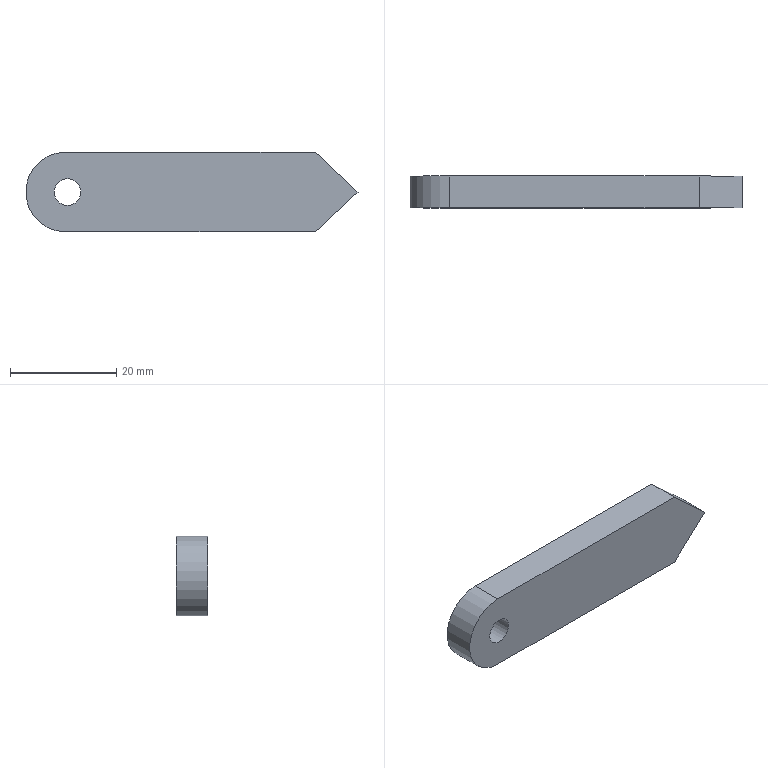Component | NX | TRI_SLIDER_2 | 1 solid | 8 faces | box 62.5 x 6 x 15 mm | volume 5000 mm3 | plane 6 | cylinder 2 | commonest cylinder face diameters 15 x1 5 x1
STEP:
#1=CARTESIAN_POINT('',(0.,0.,0.));
#2=DIRECTION('',(0.,0.,1.));
#3=DIRECTION('',(1.,0.,0.));
#4=AXIS2_PLACEMENT_3D('',#1,#2,#3);
#5=CARTESIAN_POINT('',(54.023,-12.,79.479));
#6=VERTEX_POINT('',#5);
#7=CARTESIAN_POINT('',(46.003,-12.,72.));
#8=VERTEX_POINT('',#7);
#9=CARTESIAN_POINT('',(54.023,-12.,79.479));
#10=DIRECTION('',(-0.7314,0.,-0.682));
#11=VECTOR('',#10,1.);
#12=LINE('',#9,#11);
#13=CARTESIAN_POINT('',(54.023,-18.,79.479));
#14=DIRECTION('',(0.682,0.,-0.7314));
#15=DIRECTION('',(0.7314,0.,0.682));
#16=AXIS2_PLACEMENT_3D('',#13,#14,#15);
#17=PLANE('',#16);
#18=CARTESIAN_POINT('',(0.,-6.));
#19=DIRECTION('',(-1.,0.));
#20=VECTOR('',#19,1.);
#21=LINE('',#18,#20);
#22=(GEOMETRIC_REPRESENTATION_CONTEXT(2)PARAMETRIC_REPRESENTATION_CONTEXT()REPRESENTATION_CONTEXT('',''));
#23=DEFINITIONAL_REPRESENTATION('',(#21),#22);
#24=PCURVE('',#17,#23);
#25=CARTESIAN_POINT('',(-0.9773,-12.,79.5));
#26=DIRECTION('',(0.,1.,0.));
#27=DIRECTION('',(1.,0.,0.));
#28=AXIS2_PLACEMENT_3D('',#25,#26,#27);
#29=PLANE('',#28);
#30=CARTESIAN_POINT('',(55.,0.02132));
#31=DIRECTION('',(-0.7314,0.682));
#32=VECTOR('',#31,1.);
#33=LINE('',#30,#32);
#34=(GEOMETRIC_REPRESENTATION_CONTEXT(2)PARAMETRIC_REPRESENTATION_CONTEXT()REPRESENTATION_CONTEXT('',''));
#35=DEFINITIONAL_REPRESENTATION('',(#33),#34);
#36=PCURVE('',#29,#35);
#37=SURFACE_CURVE('',#12,(#24,#36),.PCURVE_S1.);
#38=EDGE_CURVE('',#6,#8,#37,.T.);
#39=ORIENTED_EDGE('',*,*,#38,.F.);
#40=CARTESIAN_POINT('',(54.023,-18.,79.479));
#41=VERTEX_POINT('',#40);
#42=CARTESIAN_POINT('',(54.023,-18.,79.479));
#43=DIRECTION('',(0.,1.,0.));
#44=VECTOR('',#43,1.);
#45=LINE('',#42,#44);
#46=CARTESIAN_POINT('',(0.,0.));
#47=DIRECTION('',(0.,-1.));
#48=VECTOR('',#47,1.);
#49=LINE('',#46,#48);
#50=(GEOMETRIC_REPRESENTATION_CONTEXT(2)PARAMETRIC_REPRESENTATION_CONTEXT()REPRESENTATION_CONTEXT('',''));
#51=DEFINITIONAL_REPRESENTATION('',(#49),#50);
#52=PCURVE('',#17,#51);
#53=CARTESIAN_POINT('',(45.957,-18.,87.));
#54=DIRECTION('',(0.682,0.,0.7314));
#55=DIRECTION('',(-0.7314,0.,0.682));
#56=AXIS2_PLACEMENT_3D('',#53,#54,#55);
#57=PLANE('',#56);
#58=CARTESIAN_POINT('',(-11.028,0.));
#59=DIRECTION('',(0.,-1.));
#60=VECTOR('',#59,1.);
#61=LINE('',#58,#60);
#62=(GEOMETRIC_REPRESENTATION_CONTEXT(2)PARAMETRIC_REPRESENTATION_CONTEXT()REPRESENTATION_CONTEXT('',''));
#63=DEFINITIONAL_REPRESENTATION('',(#61),#62);
#64=PCURVE('',#57,#63);
#65=SURFACE_CURVE('',#45,(#52,#64),.PCURVE_S1.);
#66=EDGE_CURVE('',#41,#6,#65,.T.);
#67=ORIENTED_EDGE('',*,*,#66,.F.);
#68=CARTESIAN_POINT('',(46.003,-18.,72.));
#69=VERTEX_POINT('',#68);
#70=CARTESIAN_POINT('',(54.023,-18.,79.479));
#71=DIRECTION('',(-0.7314,0.,-0.682));
#72=VECTOR('',#71,1.);
#73=LINE('',#70,#72);
#74=CARTESIAN_POINT('',(0.,0.));
#75=DIRECTION('',(-1.,0.));
#76=VECTOR('',#75,1.);
#77=LINE('',#74,#76);
#78=(GEOMETRIC_REPRESENTATION_CONTEXT(2)PARAMETRIC_REPRESENTATION_CONTEXT()REPRESENTATION_CONTEXT('',''));
#79=DEFINITIONAL_REPRESENTATION('',(#77),#78);
#80=PCURVE('',#17,#79);
#81=CARTESIAN_POINT('',(-0.9773,-18.,79.5));
#82=DIRECTION('',(0.,1.,0.));
#83=DIRECTION('',(1.,0.,0.));
#84=AXIS2_PLACEMENT_3D('',#81,#82,#83);
#85=PLANE('',#84);
#86=CARTESIAN_POINT('',(55.,0.02132));
#87=DIRECTION('',(-0.7314,0.682));
#88=VECTOR('',#87,1.);
#89=LINE('',#86,#88);
#90=(GEOMETRIC_REPRESENTATION_CONTEXT(2)PARAMETRIC_REPRESENTATION_CONTEXT()REPRESENTATION_CONTEXT('',''));
#91=DEFINITIONAL_REPRESENTATION('',(#89),#90);
#92=PCURVE('',#85,#91);
#93=SURFACE_CURVE('',#73,(#80,#92),.PCURVE_S1.);
#94=EDGE_CURVE('',#41,#69,#93,.T.);
#95=ORIENTED_EDGE('',*,*,#94,.T.);
#96=CARTESIAN_POINT('',(46.003,-18.,72.));
#97=DIRECTION('',(0.,1.,0.));
#98=VECTOR('',#97,1.);
#99=LINE('',#96,#98);
#100=CARTESIAN_POINT('',(-10.966,0.));
#101=DIRECTION('',(0.,-1.));
#102=VECTOR('',#101,1.);
#103=LINE('',#100,#102);
#104=(GEOMETRIC_REPRESENTATION_CONTEXT(2)PARAMETRIC_REPRESENTATION_CONTEXT()REPRESENTATION_CONTEXT('',''));
#105=DEFINITIONAL_REPRESENTATION('',(#103),#104);
#106=PCURVE('',#17,#105);
#107=CARTESIAN_POINT('',(46.003,-18.,72.));
#108=DIRECTION('',(0.,0.,-1.));
#109=DIRECTION('',(1.,0.,0.));
#110=AXIS2_PLACEMENT_3D('',#107,#108,#109);
#111=PLANE('',#110);
#112=CARTESIAN_POINT('',(0.,0.));
#113=DIRECTION('',(0.,-1.));
#114=VECTOR('',#113,1.);
#115=LINE('',#112,#114);
#116=(GEOMETRIC_REPRESENTATION_CONTEXT(2)PARAMETRIC_REPRESENTATION_CONTEXT()REPRESENTATION_CONTEXT('',''));
#117=DEFINITIONAL_REPRESENTATION('',(#115),#116);
#118=PCURVE('',#111,#117);
#119=SURFACE_CURVE('',#99,(#106,#118),.PCURVE_S1.);
#120=EDGE_CURVE('',#69,#8,#119,.T.);
#121=ORIENTED_EDGE('',*,*,#120,.T.);
#122=EDGE_LOOP('',(#39,#67,#95,#121));
#123=FACE_BOUND('',#122,.T.);
#124=ADVANCED_FACE('',(#123),#17,.T.);
#125=CARTESIAN_POINT('',(-0.9773,-12.,72.));
#126=VERTEX_POINT('',#125);
#127=CARTESIAN_POINT('',(46.003,-12.,72.));
#128=DIRECTION('',(-1.,0.,-0.));
#129=VECTOR('',#128,1.);
#130=LINE('',#127,#129);
#131=CARTESIAN_POINT('',(0.,-6.));
#132=DIRECTION('',(-1.,0.));
#133=VECTOR('',#132,1.);
#134=LINE('',#131,#133);
#135=(GEOMETRIC_REPRESENTATION_CONTEXT(2)PARAMETRIC_REPRESENTATION_CONTEXT()REPRESENTATION_CONTEXT('',''));
#136=DEFINITIONAL_REPRESENTATION('',(#134),#135);
#137=PCURVE('',#111,#136);
#138=CARTESIAN_POINT('',(46.98,7.5));
#139=DIRECTION('',(-1.,0.));
#140=VECTOR('',#139,1.);
#141=LINE('',#138,#140);
#142=(GEOMETRIC_REPRESENTATION_CONTEXT(2)PARAMETRIC_REPRESENTATION_CONTEXT()REPRESENTATION_CONTEXT('',''));
#143=DEFINITIONAL_REPRESENTATION('',(#141),#142);
#144=PCURVE('',#29,#143);
#145=SURFACE_CURVE('',#130,(#137,#144),.PCURVE_S1.);
#146=EDGE_CURVE('',#8,#126,#145,.T.);
#147=ORIENTED_EDGE('',*,*,#146,.F.);
#148=ORIENTED_EDGE('',*,*,#120,.F.);
#149=CARTESIAN_POINT('',(-0.9773,-18.,72.));
#150=VERTEX_POINT('',#149);
#151=CARTESIAN_POINT('',(46.003,-18.,72.));
#152=DIRECTION('',(-1.,0.,-0.));
#153=VECTOR('',#152,1.);
#154=LINE('',#151,#153);
#155=CARTESIAN_POINT('',(0.,0.));
#156=DIRECTION('',(-1.,0.));
#157=VECTOR('',#156,1.);
#158=LINE('',#155,#157);
#159=(GEOMETRIC_REPRESENTATION_CONTEXT(2)PARAMETRIC_REPRESENTATION_CONTEXT()REPRESENTATION_CONTEXT('',''));
#160=DEFINITIONAL_REPRESENTATION('',(#158),#159);
#161=PCURVE('',#111,#160);
#162=CARTESIAN_POINT('',(46.98,7.5));
#163=DIRECTION('',(-1.,0.));
#164=VECTOR('',#163,1.);
#165=LINE('',#162,#164);
#166=(GEOMETRIC_REPRESENTATION_CONTEXT(2)PARAMETRIC_REPRESENTATION_CONTEXT()REPRESENTATION_CONTEXT('',''));
#167=DEFINITIONAL_REPRESENTATION('',(#165),#166);
#168=PCURVE('',#85,#167);
#169=SURFACE_CURVE('',#154,(#161,#168),.PCURVE_S1.);
#170=EDGE_CURVE('',#69,#150,#169,.T.);
#171=ORIENTED_EDGE('',*,*,#170,.T.);
#172=CARTESIAN_POINT('',(-0.9773,-18.,72.));
#173=DIRECTION('',(0.,1.,0.));
#174=VECTOR('',#173,1.);
#175=LINE('',#172,#174);
#176=CARTESIAN_POINT('',(-46.98,0.));
#177=DIRECTION('',(0.,-1.));
#178=VECTOR('',#177,1.);
#179=LINE('',#176,#178);
#180=(GEOMETRIC_REPRESENTATION_CONTEXT(2)PARAMETRIC_REPRESENTATION_CONTEXT()REPRESENTATION_CONTEXT('',''));
#181=DEFINITIONAL_REPRESENTATION('',(#179),#180);
#182=PCURVE('',#111,#181);
#183=CARTESIAN_POINT('',(-0.9773,-18.,79.5));
#184=DIRECTION('',(0.,1.,0.));
#185=DIRECTION('',(1.,0.,0.));
#186=AXIS2_PLACEMENT_3D('',#183,#184,#185);
#187=CYLINDRICAL_SURFACE('',#186,7.5);
#188=CARTESIAN_POINT('',(1.571,0.));
#189=DIRECTION('',(0.,1.));
#190=VECTOR('',#189,1.);
#191=LINE('',#188,#190);
#192=(GEOMETRIC_REPRESENTATION_CONTEXT(2)PARAMETRIC_REPRESENTATION_CONTEXT()REPRESENTATION_CONTEXT('',''));
#193=DEFINITIONAL_REPRESENTATION('',(#191),#192);
#194=PCURVE('',#187,#193);
#195=SURFACE_CURVE('',#175,(#182,#194),.PCURVE_S1.);
#196=EDGE_CURVE('',#150,#126,#195,.T.);
#197=ORIENTED_EDGE('',*,*,#196,.T.);
#198=EDGE_LOOP('',(#147,#148,#171,#197));
#199=FACE_BOUND('',#198,.T.);
#200=ADVANCED_FACE('',(#199),#111,.T.);
#201=CARTESIAN_POINT('',(-0.9773,-12.,87.));
#202=VERTEX_POINT('',#201);
#203=CARTESIAN_POINT('',(-0.9773,-12.,79.5));
#204=DIRECTION('',(0.,1.,0.));
#205=DIRECTION('',(-1.,0.,0.));
#206=AXIS2_PLACEMENT_3D('',#203,#204,#205);
#207=CIRCLE('',#206,7.5);
#208=CARTESIAN_POINT('',(-3.142,6.));
#209=DIRECTION('',(1.,0.));
#210=VECTOR('',#209,1.);
#211=LINE('',#208,#210);
#212=(GEOMETRIC_REPRESENTATION_CONTEXT(2)PARAMETRIC_REPRESENTATION_CONTEXT()REPRESENTATION_CONTEXT('',''));
#213=DEFINITIONAL_REPRESENTATION('',(#211),#212);
#214=PCURVE('',#187,#213);
#215=CARTESIAN_POINT('',(0.,0.));
#216=DIRECTION('',(-1.,0.));
#217=AXIS2_PLACEMENT_2D('',#215,#216);
#218=CIRCLE('',#217,7.5);
#219=(GEOMETRIC_REPRESENTATION_CONTEXT(2)PARAMETRIC_REPRESENTATION_CONTEXT()REPRESENTATION_CONTEXT('',''));
#220=DEFINITIONAL_REPRESENTATION('',(#218),#219);
#221=PCURVE('',#29,#220);
#222=SURFACE_CURVE('',#207,(#214,#221),.PCURVE_S1.);
#223=EDGE_CURVE('',#126,#202,#222,.T.);
#224=ORIENTED_EDGE('',*,*,#223,.F.);
#225=ORIENTED_EDGE('',*,*,#196,.F.);
#226=CARTESIAN_POINT('',(-0.9773,-18.,87.));
#227=VERTEX_POINT('',#226);
#228=CARTESIAN_POINT('',(-0.9773,-18.,79.5));
#229=DIRECTION('',(0.,1.,0.));
#230=DIRECTION('',(-1.,0.,0.));
#231=AXIS2_PLACEMENT_3D('',#228,#229,#230);
#232=CIRCLE('',#231,7.5);
#233=CARTESIAN_POINT('',(-3.142,0.));
#234=DIRECTION('',(1.,0.));
#235=VECTOR('',#234,1.);
#236=LINE('',#233,#235);
#237=(GEOMETRIC_REPRESENTATION_CONTEXT(2)PARAMETRIC_REPRESENTATION_CONTEXT()REPRESENTATION_CONTEXT('',''));
#238=DEFINITIONAL_REPRESENTATION('',(#236),#237);
#239=PCURVE('',#187,#238);
#240=CARTESIAN_POINT('',(0.,0.));
#241=DIRECTION('',(-1.,0.));
#242=AXIS2_PLACEMENT_2D('',#240,#241);
#243=CIRCLE('',#242,7.5);
#244=(GEOMETRIC_REPRESENTATION_CONTEXT(2)PARAMETRIC_REPRESENTATION_CONTEXT()REPRESENTATION_CONTEXT('',''));
#245=DEFINITIONAL_REPRESENTATION('',(#243),#244);
#246=PCURVE('',#85,#245);
#247=SURFACE_CURVE('',#232,(#239,#246),.PCURVE_S1.);
#248=EDGE_CURVE('',#150,#227,#247,.T.);
#249=ORIENTED_EDGE('',*,*,#248,.T.);
#250=CARTESIAN_POINT('',(-0.9773,-18.,87.));
#251=DIRECTION('',(0.,1.,0.));
#252=VECTOR('',#251,1.);
#253=LINE('',#250,#252);
#254=CARTESIAN_POINT('',(4.712,0.));
#255=DIRECTION('',(0.,1.));
#256=VECTOR('',#255,1.);
#257=LINE('',#254,#256);
#258=(GEOMETRIC_REPRESENTATION_CONTEXT(2)PARAMETRIC_REPRESENTATION_CONTEXT()REPRESENTATION_CONTEXT('',''));
#259=DEFINITIONAL_REPRESENTATION('',(#257),#258);
#260=PCURVE('',#187,#259);
#261=CARTESIAN_POINT('',(-0.9773,-18.,87.));
#262=DIRECTION('',(-0.,0.,1.));
#263=DIRECTION('',(-1.,0.,-0.));
#264=AXIS2_PLACEMENT_3D('',#261,#262,#263);
#265=PLANE('',#264);
#266=CARTESIAN_POINT('',(0.,0.));
#267=DIRECTION('',(0.,-1.));
#268=VECTOR('',#267,1.);
#269=LINE('',#266,#268);
#270=(GEOMETRIC_REPRESENTATION_CONTEXT(2)PARAMETRIC_REPRESENTATION_CONTEXT()REPRESENTATION_CONTEXT('',''));
#271=DEFINITIONAL_REPRESENTATION('',(#269),#270);
#272=PCURVE('',#265,#271);
#273=SURFACE_CURVE('',#253,(#260,#272),.PCURVE_S1.);
#274=EDGE_CURVE('',#227,#202,#273,.T.);
#275=ORIENTED_EDGE('',*,*,#274,.T.);
#276=EDGE_LOOP('',(#224,#225,#249,#275));
#277=FACE_BOUND('',#276,.T.);
#278=ADVANCED_FACE('',(#277),#187,.T.);
#279=CARTESIAN_POINT('',(45.957,-12.,87.));
#280=VERTEX_POINT('',#279);
#281=CARTESIAN_POINT('',(-0.9773,-12.,87.));
#282=DIRECTION('',(1.,0.,0.));
#283=VECTOR('',#282,1.);
#284=LINE('',#281,#283);
#285=CARTESIAN_POINT('',(0.,-6.));
#286=DIRECTION('',(-1.,0.));
#287=VECTOR('',#286,1.);
#288=LINE('',#285,#287);
#289=(GEOMETRIC_REPRESENTATION_CONTEXT(2)PARAMETRIC_REPRESENTATION_CONTEXT()REPRESENTATION_CONTEXT('',''));
#290=DEFINITIONAL_REPRESENTATION('',(#288),#289);
#291=PCURVE('',#265,#290);
#292=CARTESIAN_POINT('',(0.,-7.5));
#293=DIRECTION('',(1.,-0.));
#294=VECTOR('',#293,1.);
#295=LINE('',#292,#294);
#296=(GEOMETRIC_REPRESENTATION_CONTEXT(2)PARAMETRIC_REPRESENTATION_CONTEXT()REPRESENTATION_CONTEXT('',''));
#297=DEFINITIONAL_REPRESENTATION('',(#295),#296);
#298=PCURVE('',#29,#297);
#299=SURFACE_CURVE('',#284,(#291,#298),.PCURVE_S1.);
#300=EDGE_CURVE('',#202,#280,#299,.T.);
#301=ORIENTED_EDGE('',*,*,#300,.F.);
#302=ORIENTED_EDGE('',*,*,#274,.F.);
#303=CARTESIAN_POINT('',(45.957,-18.,87.));
#304=VERTEX_POINT('',#303);
#305=CARTESIAN_POINT('',(-0.9773,-18.,87.));
#306=DIRECTION('',(1.,0.,0.));
#307=VECTOR('',#306,1.);
#308=LINE('',#305,#307);
#309=CARTESIAN_POINT('',(0.,0.));
#310=DIRECTION('',(-1.,0.));
#311=VECTOR('',#310,1.);
#312=LINE('',#309,#311);
#313=(GEOMETRIC_REPRESENTATION_CONTEXT(2)PARAMETRIC_REPRESENTATION_CONTEXT()REPRESENTATION_CONTEXT('',''));
#314=DEFINITIONAL_REPRESENTATION('',(#312),#313);
#315=PCURVE('',#265,#314);
#316=CARTESIAN_POINT('',(0.,-7.5));
#317=DIRECTION('',(1.,-0.));
#318=VECTOR('',#317,1.);
#319=LINE('',#316,#318);
#320=(GEOMETRIC_REPRESENTATION_CONTEXT(2)PARAMETRIC_REPRESENTATION_CONTEXT()REPRESENTATION_CONTEXT('',''));
#321=DEFINITIONAL_REPRESENTATION('',(#319),#320);
#322=PCURVE('',#85,#321);
#323=SURFACE_CURVE('',#308,(#315,#322),.PCURVE_S1.);
#324=EDGE_CURVE('',#227,#304,#323,.T.);
#325=ORIENTED_EDGE('',*,*,#324,.T.);
#326=CARTESIAN_POINT('',(45.957,-18.,87.));
#327=DIRECTION('',(0.,1.,0.));
#328=VECTOR('',#327,1.);
#329=LINE('',#326,#328);
#330=CARTESIAN_POINT('',(-46.934,0.));
#331=DIRECTION('',(0.,-1.));
#332=VECTOR('',#331,1.);
#333=LINE('',#330,#332);
#334=(GEOMETRIC_REPRESENTATION_CONTEXT(2)PARAMETRIC_REPRESENTATION_CONTEXT()REPRESENTATION_CONTEXT('',''));
#335=DEFINITIONAL_REPRESENTATION('',(#333),#334);
#336=PCURVE('',#265,#335);
#337=CARTESIAN_POINT('',(0.,0.));
#338=DIRECTION('',(0.,-1.));
#339=VECTOR('',#338,1.);
#340=LINE('',#337,#339);
#341=(GEOMETRIC_REPRESENTATION_CONTEXT(2)PARAMETRIC_REPRESENTATION_CONTEXT()REPRESENTATION_CONTEXT('',''));
#342=DEFINITIONAL_REPRESENTATION('',(#340),#341);
#343=PCURVE('',#57,#342);
#344=SURFACE_CURVE('',#329,(#336,#343),.PCURVE_S1.);
#345=EDGE_CURVE('',#304,#280,#344,.T.);
#346=ORIENTED_EDGE('',*,*,#345,.T.);
#347=EDGE_LOOP('',(#301,#302,#325,#346));
#348=FACE_BOUND('',#347,.T.);
#349=ADVANCED_FACE('',(#348),#265,.T.);
#350=CARTESIAN_POINT('',(45.957,-12.,87.));
#351=DIRECTION('',(0.7314,0.,-0.682));
#352=VECTOR('',#351,1.);
#353=LINE('',#350,#352);
#354=CARTESIAN_POINT('',(0.,-6.));
#355=DIRECTION('',(-1.,0.));
#356=VECTOR('',#355,1.);
#357=LINE('',#354,#356);
#358=(GEOMETRIC_REPRESENTATION_CONTEXT(2)PARAMETRIC_REPRESENTATION_CONTEXT()REPRESENTATION_CONTEXT('',''));
#359=DEFINITIONAL_REPRESENTATION('',(#357),#358);
#360=PCURVE('',#57,#359);
#361=CARTESIAN_POINT('',(46.934,-7.5));
#362=DIRECTION('',(0.7314,0.682));
#363=VECTOR('',#362,1.);
#364=LINE('',#361,#363);
#365=(GEOMETRIC_REPRESENTATION_CONTEXT(2)PARAMETRIC_REPRESENTATION_CONTEXT()REPRESENTATION_CONTEXT('',''));
#366=DEFINITIONAL_REPRESENTATION('',(#364),#365);
#367=PCURVE('',#29,#366);
#368=SURFACE_CURVE('',#353,(#360,#367),.PCURVE_S1.);
#369=EDGE_CURVE('',#280,#6,#368,.T.);
#370=ORIENTED_EDGE('',*,*,#369,.F.);
#371=ORIENTED_EDGE('',*,*,#345,.F.);
#372=CARTESIAN_POINT('',(45.957,-18.,87.));
#373=DIRECTION('',(0.7314,0.,-0.682));
#374=VECTOR('',#373,1.);
#375=LINE('',#372,#374);
#376=CARTESIAN_POINT('',(0.,0.));
#377=DIRECTION('',(-1.,0.));
#378=VECTOR('',#377,1.);
#379=LINE('',#376,#378);
#380=(GEOMETRIC_REPRESENTATION_CONTEXT(2)PARAMETRIC_REPRESENTATION_CONTEXT()REPRESENTATION_CONTEXT('',''));
#381=DEFINITIONAL_REPRESENTATION('',(#379),#380);
#382=PCURVE('',#57,#381);
#383=CARTESIAN_POINT('',(46.934,-7.5));
#384=DIRECTION('',(0.7314,0.682));
#385=VECTOR('',#384,1.);
#386=LINE('',#383,#385);
#387=(GEOMETRIC_REPRESENTATION_CONTEXT(2)PARAMETRIC_REPRESENTATION_CONTEXT()REPRESENTATION_CONTEXT('',''));
#388=DEFINITIONAL_REPRESENTATION('',(#386),#387);
#389=PCURVE('',#85,#388);
#390=SURFACE_CURVE('',#375,(#382,#389),.PCURVE_S1.);
#391=EDGE_CURVE('',#304,#41,#390,.T.);
#392=ORIENTED_EDGE('',*,*,#391,.T.);
#393=ORIENTED_EDGE('',*,*,#66,.T.);
#394=EDGE_LOOP('',(#370,#371,#392,#393));
#395=FACE_BOUND('',#394,.T.);
#396=ADVANCED_FACE('',(#395),#57,.T.);
#397=CARTESIAN_POINT('',(-3.117,-18.,79.479));
#398=VERTEX_POINT('',#397);
#399=CARTESIAN_POINT('',(-0.6173,-18.,79.479));
#400=DIRECTION('',(0.,-1.,0.));
#401=DIRECTION('',(-1.,0.,0.));
#402=AXIS2_PLACEMENT_3D('',#399,#400,#401);
#403=CIRCLE('',#402,2.5);
#404=CARTESIAN_POINT('',(-0.6173,-18.,79.479));
#405=DIRECTION('',(0.,1.,0.));
#406=DIRECTION('',(1.,0.,0.));
#407=AXIS2_PLACEMENT_3D('',#404,#405,#406);
#408=CYLINDRICAL_SURFACE('',#407,2.5);
#409=CARTESIAN_POINT('',(9.425,0.));
#410=DIRECTION('',(-1.,0.));
#411=VECTOR('',#410,1.);
#412=LINE('',#409,#411);
#413=(GEOMETRIC_REPRESENTATION_CONTEXT(2)PARAMETRIC_REPRESENTATION_CONTEXT()REPRESENTATION_CONTEXT('',''));
#414=DEFINITIONAL_REPRESENTATION('',(#412),#413);
#415=PCURVE('',#408,#414);
#416=CARTESIAN_POINT('',(-2.14,0.02132));
#417=CARTESIAN_POINT('',(-2.14,4.351));
#418=CARTESIAN_POINT('',(1.61,2.186));
#419=CARTESIAN_POINT('',(5.36,0.02132));
#420=CARTESIAN_POINT('',(1.61,-2.144));
#421=CARTESIAN_POINT('',(-2.14,-4.309));
#422=CARTESIAN_POINT('',(-2.14,0.02132));
#423=(BOUNDED_CURVE()B_SPLINE_CURVE(2,(#416,#417,#418,#419,#420,#421,#422),.UNSPECIFIED.,.T.,.F.)B_SPLINE_CURVE_WITH_KNOTS((1,2,2,2,2,1),(-2.094,0.,2.094,4.189,6.283,8.378),.UNSPECIFIED.)CURVE()GEOMETRIC_REPRESENTATION_ITEM()RATIONAL_B_SPLINE_CURVE((1.,0.5,1.,0.5,1.,0.5,1.))REPRESENTATION_ITEM(''));
#424=(GEOMETRIC_REPRESENTATION_CONTEXT(2)PARAMETRIC_REPRESENTATION_CONTEXT()REPRESENTATION_CONTEXT('',''));
#425=DEFINITIONAL_REPRESENTATION('',(#423),#424);
#426=PCURVE('',#85,#425);
#427=SURFACE_CURVE('',#403,(#415,#426),.PCURVE_S1.);
#428=EDGE_CURVE('',#398,#398,#427,.T.);
#429=ORIENTED_EDGE('',*,*,#428,.F.);
#430=CARTESIAN_POINT('',(-3.117,-12.,79.479));
#431=VERTEX_POINT('',#430);
#432=CARTESIAN_POINT('',(-3.117,-18.,79.479));
#433=CARTESIAN_POINT('',(-3.117,-12.,79.479));
#434=B_SPLINE_CURVE_WITH_KNOTS('',1,(#432,#433),.UNSPECIFIED.,.F.,.F.,(2,2),(0.,6.),.PIECEWISE_BEZIER_KNOTS.);
#435=CARTESIAN_POINT('',(9.425,0.));
#436=DIRECTION('',(0.,1.));
#437=VECTOR('',#436,1.);
#438=LINE('',#435,#437);
#439=(GEOMETRIC_REPRESENTATION_CONTEXT(2)PARAMETRIC_REPRESENTATION_CONTEXT()REPRESENTATION_CONTEXT('',''));
#440=DEFINITIONAL_REPRESENTATION('',(#438),#439);
#441=PCURVE('',#408,#440);
#442=CARTESIAN_POINT('',(3.142,0.));
#443=DIRECTION('',(0.,1.));
#444=VECTOR('',#443,1.);
#445=LINE('',#442,#444);
#446=(GEOMETRIC_REPRESENTATION_CONTEXT(2)PARAMETRIC_REPRESENTATION_CONTEXT()REPRESENTATION_CONTEXT('',''));
#447=DEFINITIONAL_REPRESENTATION('',(#445),#446);
#448=PCURVE('',#408,#447);
#449=SEAM_CURVE('',#434,(#441,#448),.PCURVE_S1.);
#450=EDGE_CURVE('',#398,#431,#449,.T.);
#451=ORIENTED_EDGE('',*,*,#450,.T.);
#452=CARTESIAN_POINT('',(-0.6173,-12.,79.479));
#453=DIRECTION('',(0.,-1.,0.));
#454=DIRECTION('',(-1.,0.,0.));
#455=AXIS2_PLACEMENT_3D('',#452,#453,#454);
#456=CIRCLE('',#455,2.5);
#457=CARTESIAN_POINT('',(9.425,6.));
#458=DIRECTION('',(-1.,0.));
#459=VECTOR('',#458,1.);
#460=LINE('',#457,#459);
#461=(GEOMETRIC_REPRESENTATION_CONTEXT(2)PARAMETRIC_REPRESENTATION_CONTEXT()REPRESENTATION_CONTEXT('',''));
#462=DEFINITIONAL_REPRESENTATION('',(#460),#461);
#463=PCURVE('',#408,#462);
#464=CARTESIAN_POINT('',(-2.14,0.02132));
#465=CARTESIAN_POINT('',(-2.14,4.351));
#466=CARTESIAN_POINT('',(1.61,2.186));
#467=CARTESIAN_POINT('',(5.36,0.02132));
#468=CARTESIAN_POINT('',(1.61,-2.144));
#469=CARTESIAN_POINT('',(-2.14,-4.309));
#470=CARTESIAN_POINT('',(-2.14,0.02132));
#471=(BOUNDED_CURVE()B_SPLINE_CURVE(2,(#464,#465,#466,#467,#468,#469,#470),.UNSPECIFIED.,.T.,.F.)B_SPLINE_CURVE_WITH_KNOTS((1,2,2,2,2,1),(-2.094,0.,2.094,4.189,6.283,8.378),.UNSPECIFIED.)CURVE()GEOMETRIC_REPRESENTATION_ITEM()RATIONAL_B_SPLINE_CURVE((1.,0.5,1.,0.5,1.,0.5,1.))REPRESENTATION_ITEM(''));
#472=(GEOMETRIC_REPRESENTATION_CONTEXT(2)PARAMETRIC_REPRESENTATION_CONTEXT()REPRESENTATION_CONTEXT('',''));
#473=DEFINITIONAL_REPRESENTATION('',(#471),#472);
#474=PCURVE('',#29,#473);
#475=SURFACE_CURVE('',#456,(#463,#474),.PCURVE_S1.);
#476=EDGE_CURVE('',#431,#431,#475,.T.);
#477=ORIENTED_EDGE('',*,*,#476,.T.);
#478=ORIENTED_EDGE('',*,*,#450,.F.);
#479=EDGE_LOOP('',(#429,#451,#477,#478));
#480=FACE_BOUND('',#479,.F.);
#481=ADVANCED_FACE('',(#480),#408,.F.);
#482=ORIENTED_EDGE('',*,*,#94,.F.);
#483=ORIENTED_EDGE('',*,*,#391,.F.);
#484=ORIENTED_EDGE('',*,*,#324,.F.);
#485=ORIENTED_EDGE('',*,*,#248,.F.);
#486=ORIENTED_EDGE('',*,*,#170,.F.);
#487=EDGE_LOOP('',(#482,#483,#484,#485,#486));
#488=FACE_BOUND('',#487,.T.);
#489=ORIENTED_EDGE('',*,*,#428,.F.);
#490=EDGE_LOOP('',(#489));
#491=FACE_BOUND('',#490,.T.);
#492=ADVANCED_FACE('',(#488,#491),#85,.F.);
#493=ORIENTED_EDGE('',*,*,#38,.T.);
#494=ORIENTED_EDGE('',*,*,#146,.T.);
#495=ORIENTED_EDGE('',*,*,#223,.T.);
#496=ORIENTED_EDGE('',*,*,#300,.T.);
#497=ORIENTED_EDGE('',*,*,#369,.T.);
#498=EDGE_LOOP('',(#493,#494,#495,#496,#497));
#499=FACE_BOUND('',#498,.T.);
#500=ORIENTED_EDGE('',*,*,#476,.T.);
#501=EDGE_LOOP('',(#500));
#502=FACE_BOUND('',#501,.T.);
#503=ADVANCED_FACE('',(#499,#502),#29,.T.);
#504=CLOSED_SHELL('',(#124,#200,#278,#349,#396,#481,#492,#503));
#505=MANIFOLD_SOLID_BREP('',#504);
#506=(LENGTH_UNIT()NAMED_UNIT(*)SI_UNIT(.MILLI.,.METRE.));
#507=UNCERTAINTY_MEASURE_WITH_UNIT(LENGTH_MEASURE(0.000001),#506,'','');
#508=(NAMED_UNIT(*)PLANE_ANGLE_UNIT()SI_UNIT($,.RADIAN.));
#509=(NAMED_UNIT(*)SI_UNIT($,.STERADIAN.)SOLID_ANGLE_UNIT());
#510=(GEOMETRIC_REPRESENTATION_CONTEXT(3)GLOBAL_UNCERTAINTY_ASSIGNED_CONTEXT((#507))GLOBAL_UNIT_ASSIGNED_CONTEXT((#506,#508,#509))REPRESENTATION_CONTEXT('',''));
#511=ADVANCED_BREP_SHAPE_REPRESENTATION('',(#4,#505),#510);